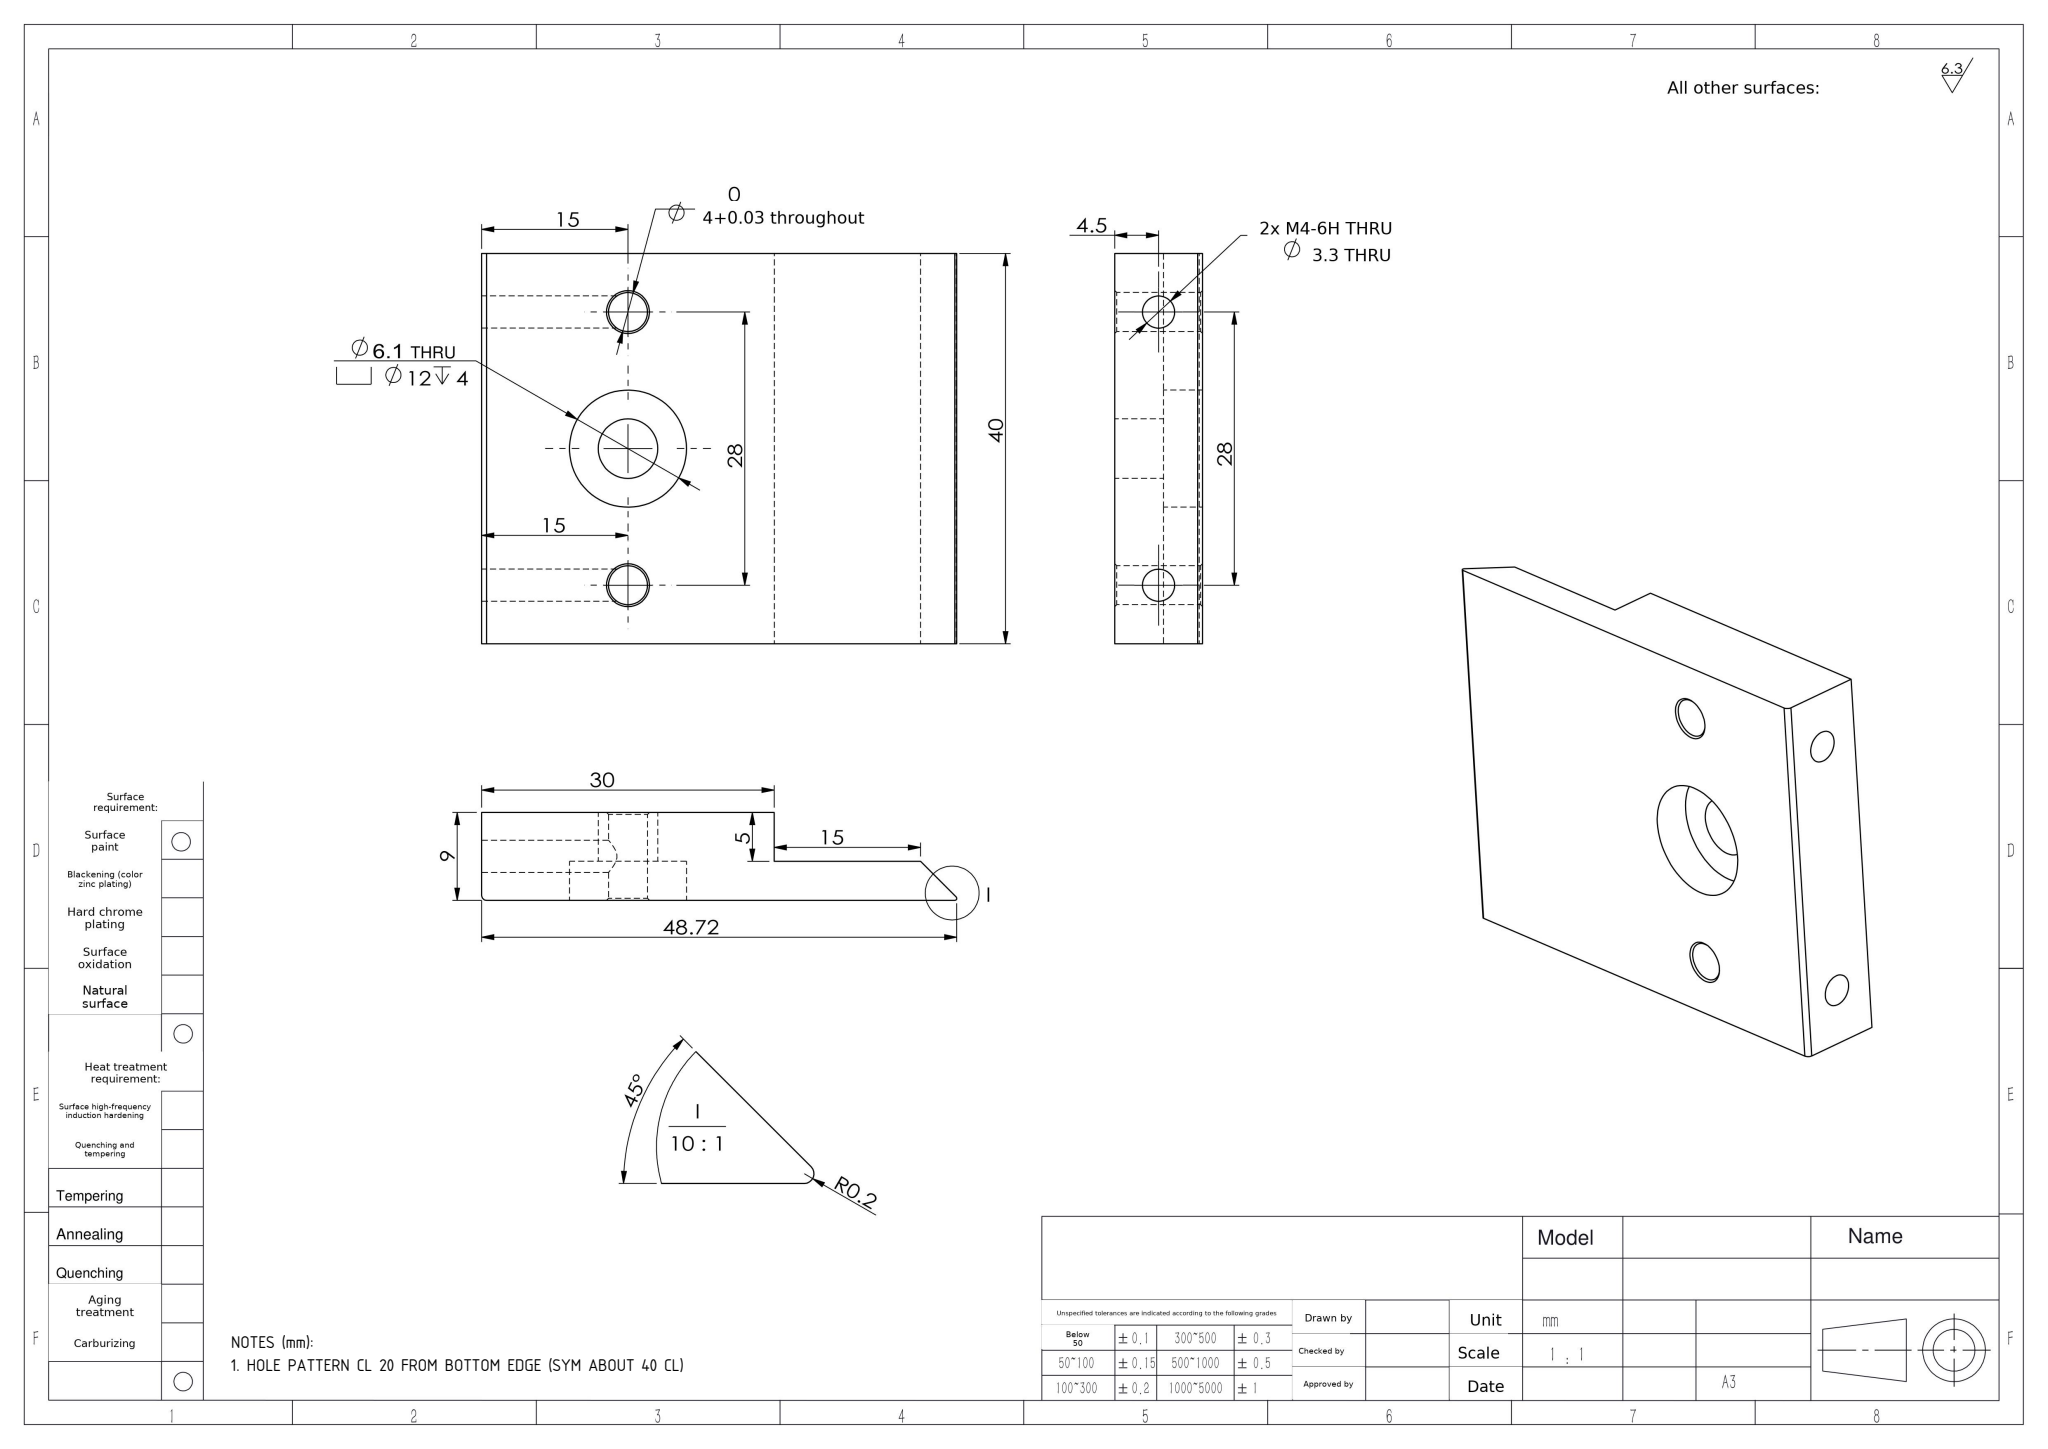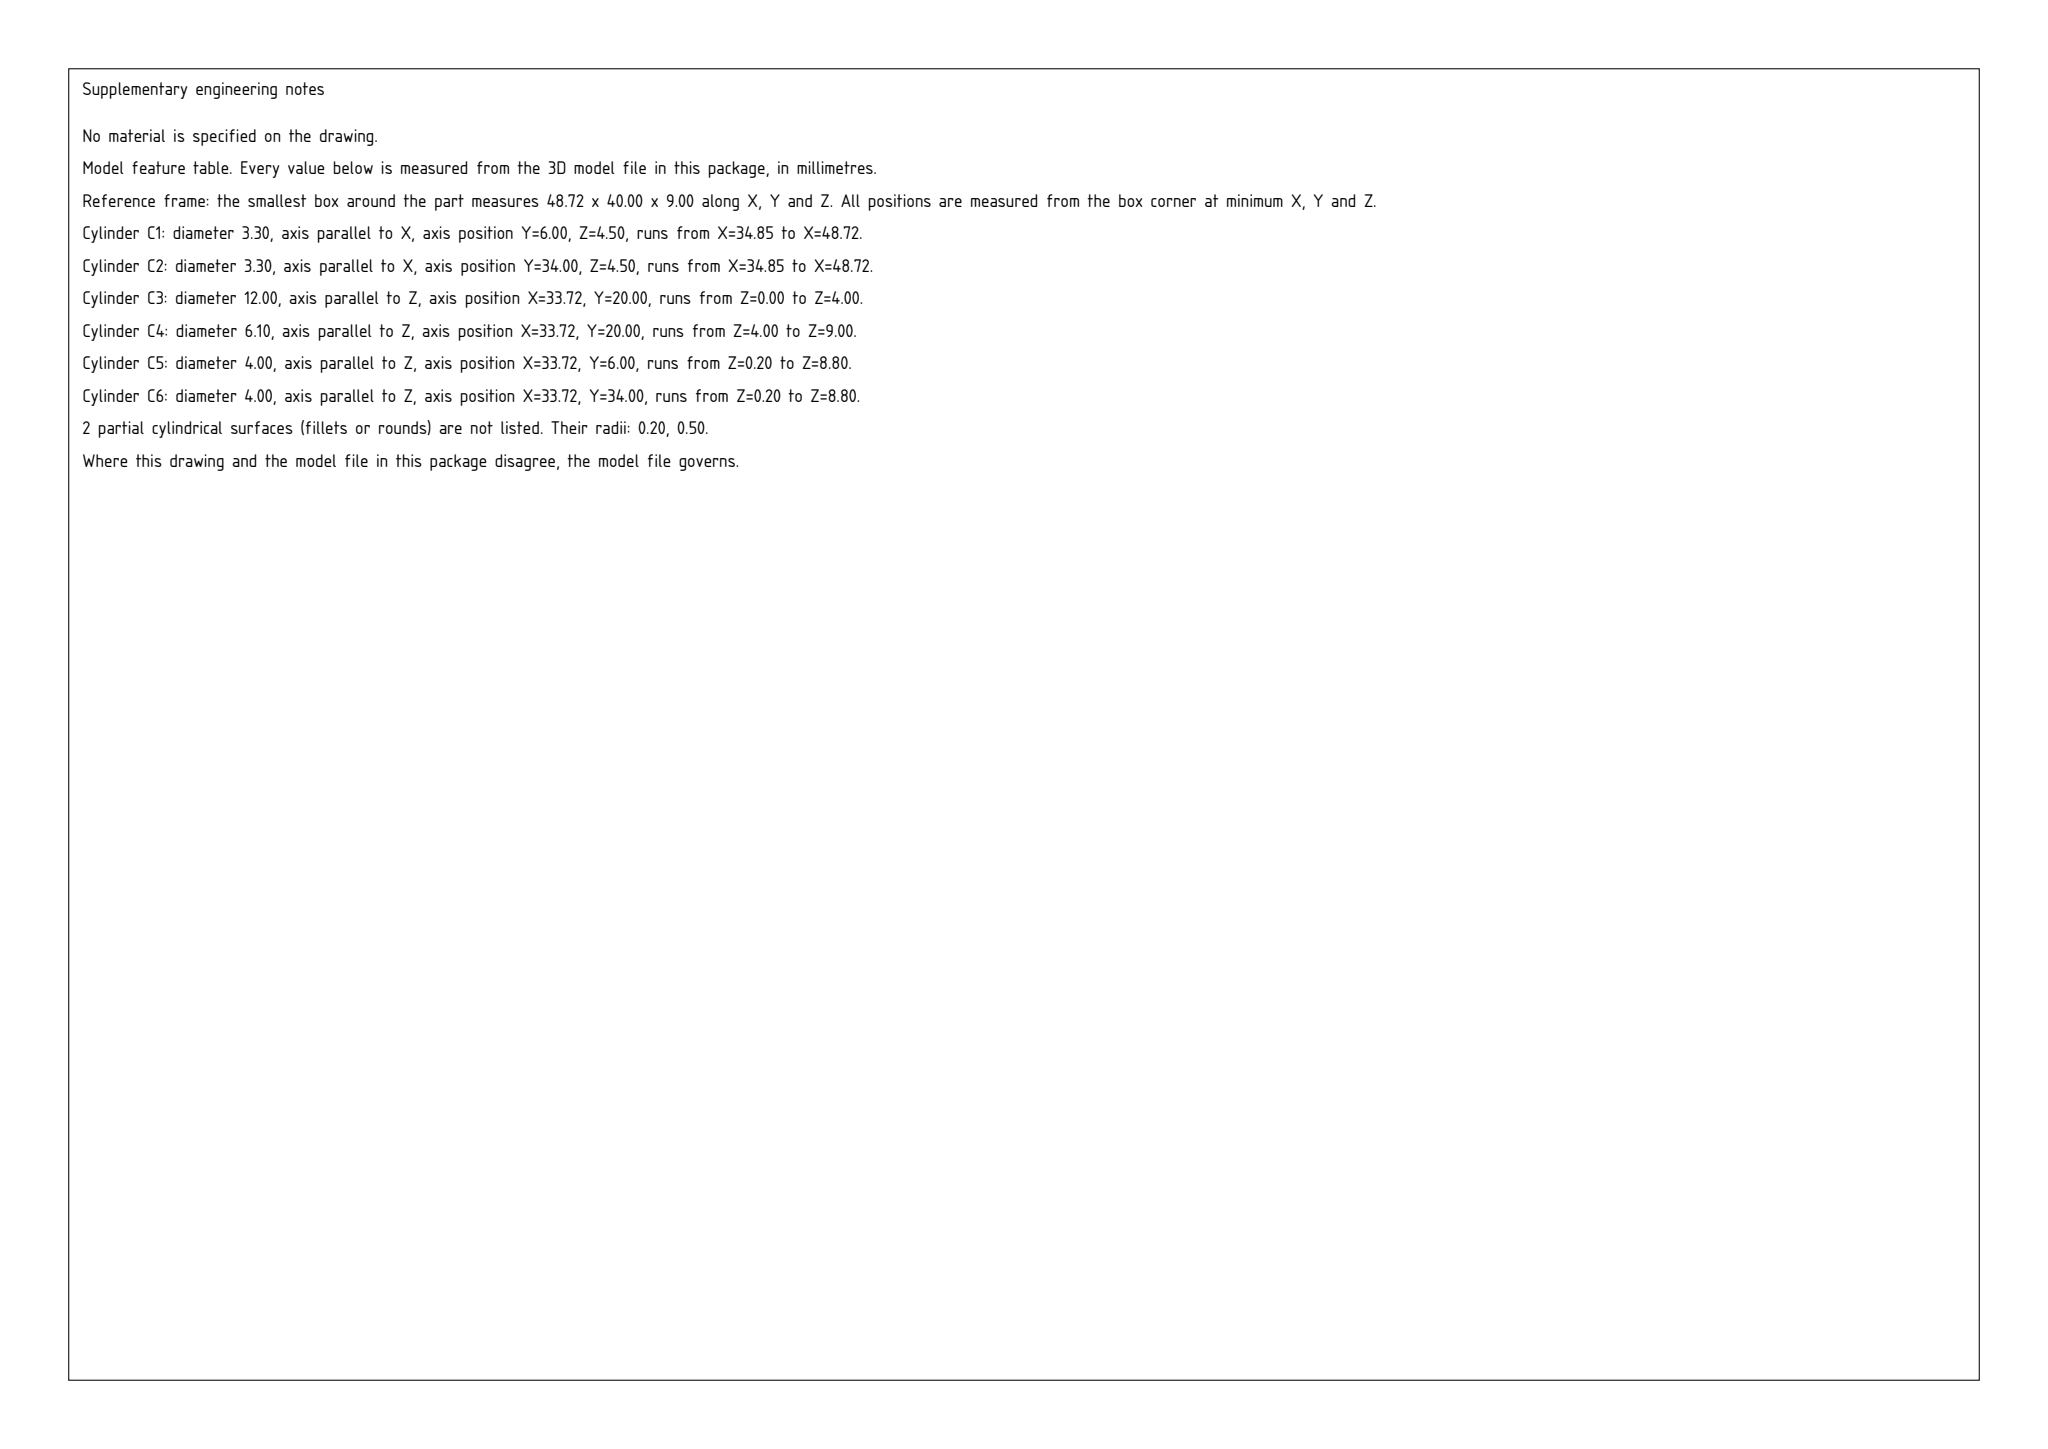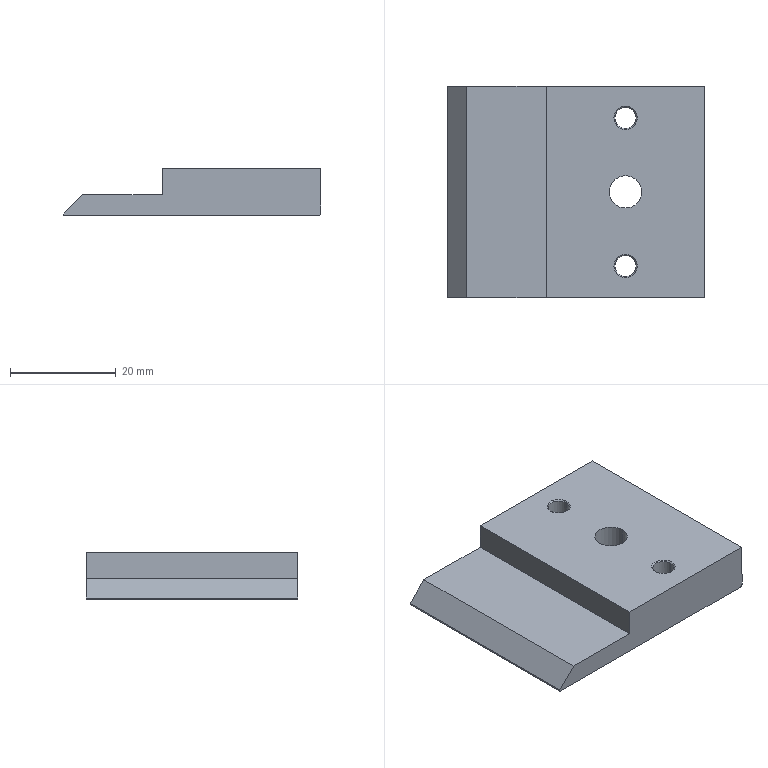Part | SolidWorks | mm | 1 solid | 31 faces | box 48.72 x 40 x 9 mm | volume 12465 mm3 | cylinder 14 | plane 9 | cone 8 | commonest cylinder face diameters 3.3 x4 4 x4 12 x2 6.1 x2 1 x1 0.4 x1
Drawing notes:
HOLE PATTERN CL 20 FROM BOTTOM EDGE (SYM ABOUT 40 CL) | from the solid: Plate height 40; outer holes at 28 spacing centered => hole CL at 20 from each 40 mm edge; Ø6.1/Ø12 C'BORE on same CL
build123d program:
from build123d import *

# Parameters (mm, degrees)
BOSS_EXTRUDE1_DEPTH        = 40
SKETCH2_W                  = 30
SKETCH2_H                  = 40
BOSS_EXTRUDE2_DEPTH        = 5
F_5_1_5_1_DIAMETER_HOLE1_D = 6.1
F_4_0_4_DIAMETER_HOLE1_D   = 4
F_4_0_4_DIAMETER_HOLE2_D   = 4
M4_TAPPED_HOLE1_REACH      = 55.684
M4_TAPPED_HOLE1_BORE_R     = 1.65
CHAMFER1_SIZE              = 0.2
FILLET1_R                  = 0.5
SKETCH12_R                 = 6
CUT_EXTRUDE2_DEPTH         = 4
FILLET2_R                  = 0.2


with BuildPart() as part:
    # Sketch1 → Boss-Extrude1 (new body)
    with BuildSketch(Plane.XZ.offset(20)):
        Polygon((49, 0), (49, 4), (4, 4), (0, 0), align=None)
    extrude(amount=-BOSS_EXTRUDE1_DEPTH)

    # Sketch2 → Boss-Extrude2 (add)
    with BuildSketch(Plane.XY.offset(4)):
        with Locations((34, 0)):
            Rectangle(SKETCH2_W, SKETCH2_H)
    extrude(amount=BOSS_EXTRUDE2_DEPTH)

    # 5.1 _5.1_ Diameter Hole1 (through all)
    with Locations(Plane(origin=(0, 0, 0), x_dir=(-1, 0, 0), z_dir=(0, 0, -1))):
        with Locations((-34, 0)):
            Hole(F_5_1_5_1_DIAMETER_HOLE1_D / 2)

    # 4.0 _4_ Diameter Hole1 (through all)
    with Locations(Plane(origin=(0, 0, 0), x_dir=(-1, 0, 0), z_dir=(0, 0, -1))):
        with Locations((-34, 14)):
            Hole(F_4_0_4_DIAMETER_HOLE1_D / 2)

    # 4.0 _4_ Diameter Hole2 (through all)
    with Locations(Plane.XY.offset(9)):
        with Locations((34, -14)):
            Hole(F_4_0_4_DIAMETER_HOLE2_D / 2)

    # M4 Tapped Hole1 bore → M4 Tapped Hole1 (cut, up to next)
    with BuildSketch(Plane(origin=(49, 0, 0), x_dir=(0, 0, -1), z_dir=(1, 0, 0)), mode=Mode.PRIVATE) as m4_tapped_hole1_sk1:
        with Locations((-4.5, -14)):
            Circle(M4_TAPPED_HOLE1_BORE_R)
    m4_tapped_hole1_tool1 = extrude(m4_tapped_hole1_sk1.sketch, amount=-M4_TAPPED_HOLE1_REACH, mode=Mode.PRIVATE) & part.part
    # M4 Tapped Hole1 bore → M4 Tapped Hole1 (cut, up to next)
    with BuildSketch(Plane(origin=(49, 0, 0), x_dir=(0, 0, -1), z_dir=(1, 0, 0)), mode=Mode.PRIVATE) as m4_tapped_hole1_sk2:
        with Locations((-4.5, 14)):
            Circle(M4_TAPPED_HOLE1_BORE_R)
    m4_tapped_hole1_tool2 = extrude(m4_tapped_hole1_sk2.sketch, amount=-M4_TAPPED_HOLE1_REACH, mode=Mode.PRIVATE) & part.part
    add(m4_tapped_hole1_tool1.solids().sort_by_distance((49, -14, 4.5))[0], mode=Mode.SUBTRACT)
    add(m4_tapped_hole1_tool2.solids().sort_by_distance((49, 14, 4.5))[0], mode=Mode.SUBTRACT)

    # Chamfer1
    chamfer1_edges = [part.edges().sort_by_distance(p)[0] for p in [
        (32, 14, 0),
        (32, 14, 9),
        (36, -14, 9),
        (36, -14, 0),
    ]]
    chamfer(chamfer1_edges, length=CHAMFER1_SIZE)

    # Fillet1
    fillet1_edges = [part.edges().sort_by_distance(p)[0] for p in [
        (49, 0, 0),
    ]]
    fillet(fillet1_edges, radius=FILLET1_R)

    # Sketch12 → Cut-Extrude2 (cut)
    with BuildSketch(Plane(origin=(0, 0, 0), x_dir=(-1, 0, 0), z_dir=(0, 0, -1))):
        with Locations((-34, 0)):
            Circle(SKETCH12_R)
    extrude(amount=-CUT_EXTRUDE2_DEPTH, mode=Mode.SUBTRACT)

    # Fillet2
    fillet2_edges = [part.edges().sort_by_distance(p)[0] for p in [
        (0, 0, 0),
    ]]
    fillet(fillet2_edges, radius=FILLET2_R)


solid = part.part